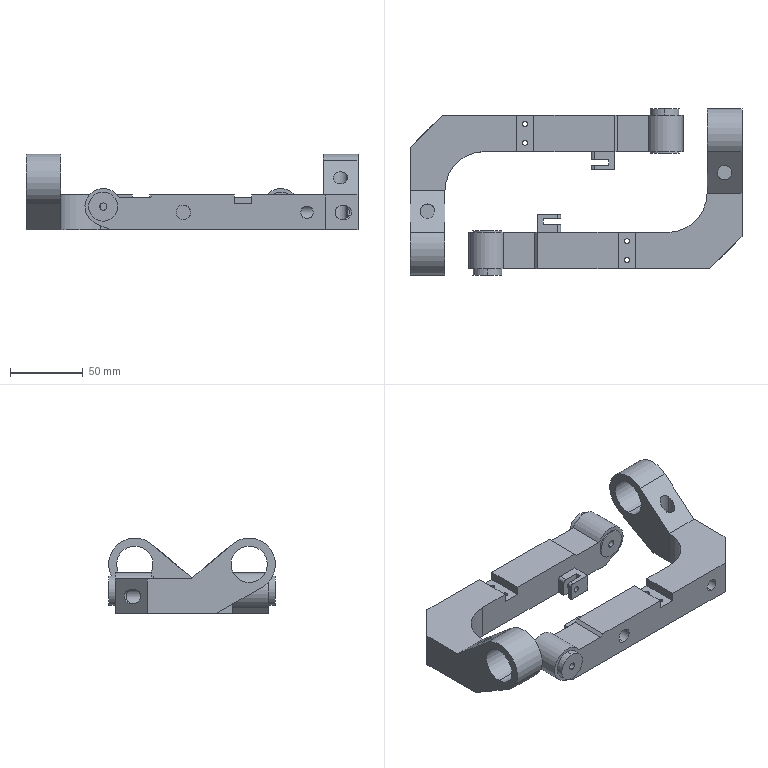CAM job | Mastercam | mm | 3 operations | part box 228 x 114.5 x 52.07
1. Facing | 24 - 100 平底刀
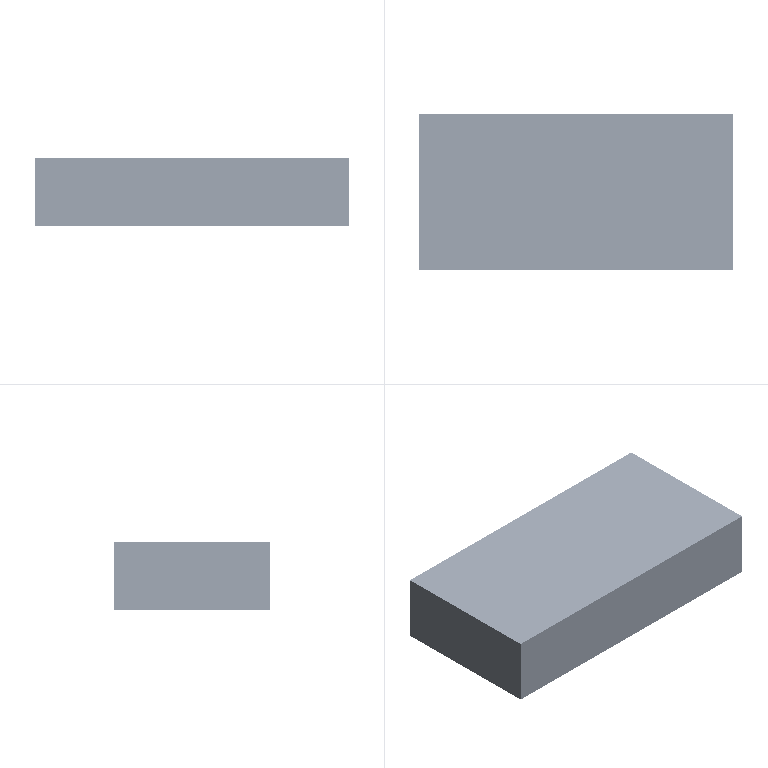2. 2D High Speed (2D Dynamic Mill) | 16 - 16 平底刀
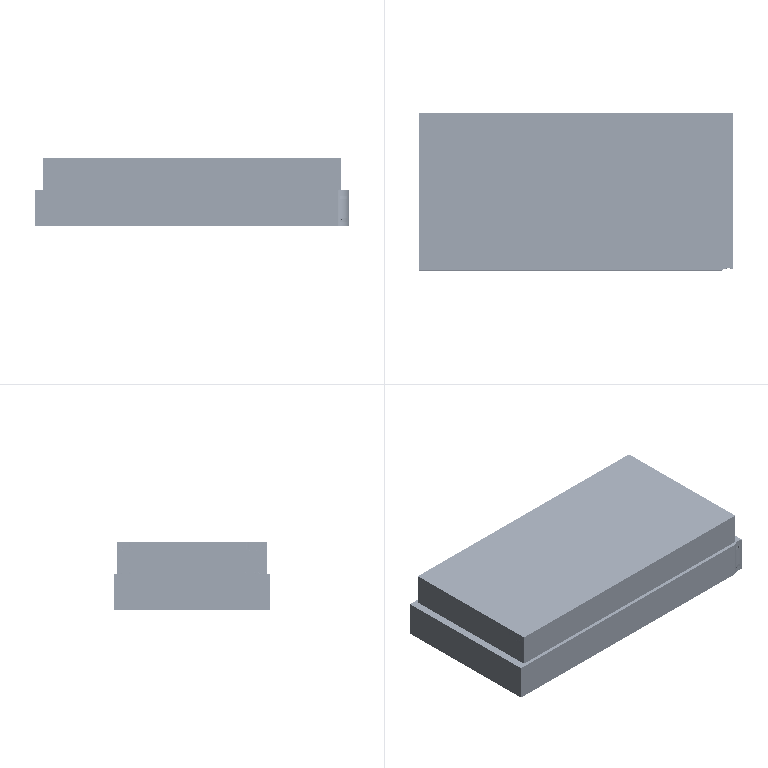3. Contour (2D) | 16 - 16 平底刀